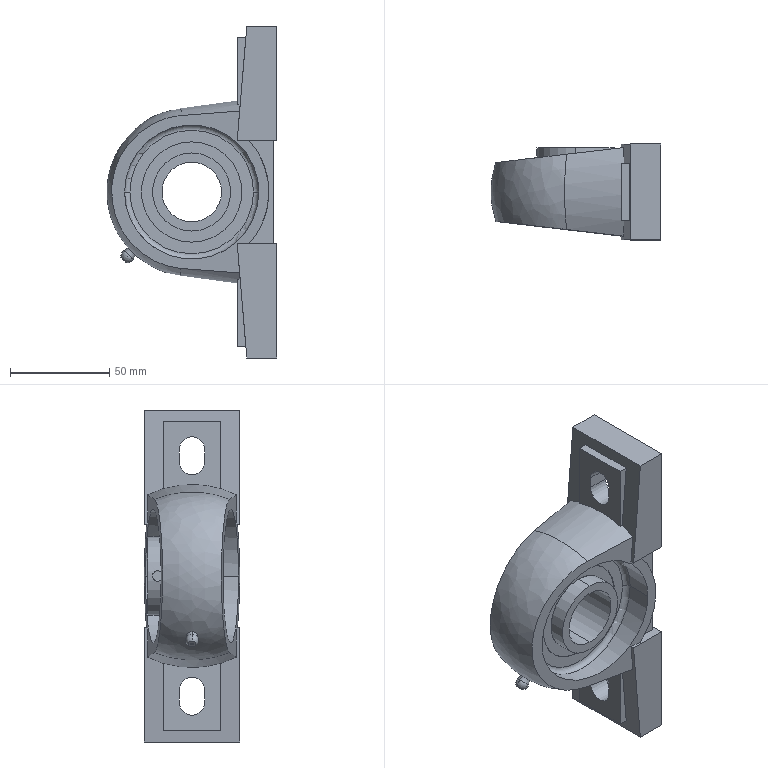Component | SolidWorks | GB_T7810-1995BearingUnitUCP206-3 | 1 solid | 121 faces | volume 196512 mm3 | plane 58 | cylinder 28 | cone 16 | sphere 8 | torus 8 | spline 3 | commonest cylinder face diameters 67.524 x6 39.28 x6 50.52 x6 13 x4 5.351 x2 30 x2 77.659 x2